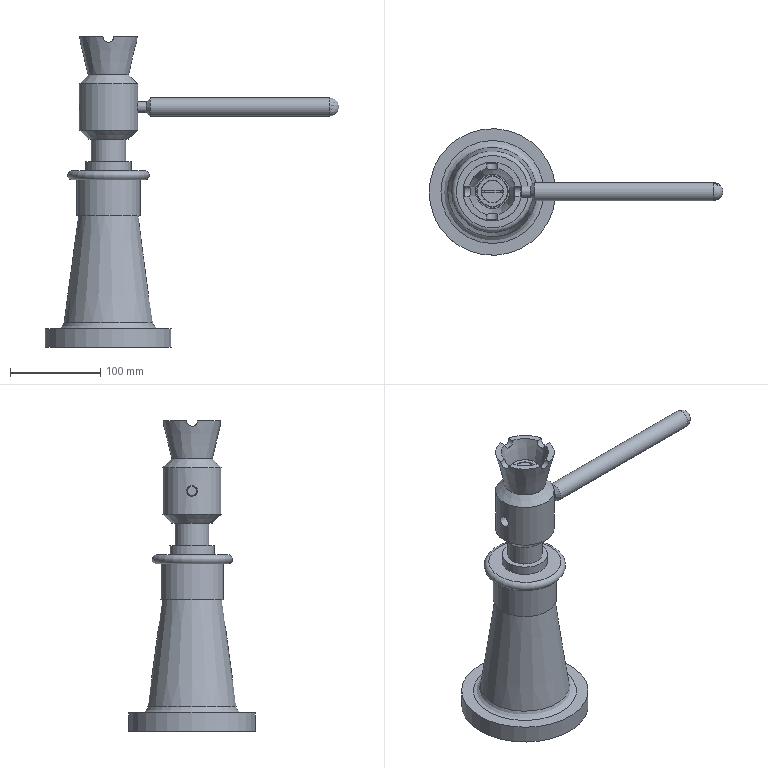Assembly | NX | mm | 7 component files | 7 solids | 67 faces | box 325 x 140 x 343 mm | volume 1154943 mm3 | plane 28 | cylinder 22 | cone 13 | torus 3 | sphere 1 | commonest cylinder face diameters 12 x6 50 x3 38 x2 10.3 x2 20 x1 100 x1 140 x1 70 x1
Bill of materials:
unnamed part 1 | 1 |  | Thick-walled hollow cup tapered like a frustum, wider at the open top. The top rim has four evenly spaced semicircular notches, and the bottom wall has a central through-hole.
unnamed part 2 | 1 |  | Stepped turned pin: a long plain cylindrical shank with a larger cylindrical collar or head that has chamfered edges on both sides. The head has a small radial cross-hole, and a small cylindrical spigot sticks out from the top face.
unnamed part 3 | 1 |  | Slender stepped cylindrical rod: a short smaller-diameter section at one end, a short chamfer or step, then a longer main body that ends in a rounded, roughly hemispherical tip.
unnamed part 4 | 1 |  | Flanged tubular bushing or grommet: a straight cylindrical sleeve with a central through-bore and a thin circular flange with rounded edges around its middle.
unnamed part 5 | 1 |  | Hollow tapered body standing on a flat circular base flange. A conical frustum rises from the flange with a fillet at its root and steps into a short cylindrical neck at the top. A through-bore runs along the axis.
unnamed part 6 | 1 |  | Slotted countersunk-head screw-like part: a conical flat-top head with a straight slot across it, a plain cylindrical shank, and a chamfered tip.
unnamed part 7 | 1 |  | Countersunk ring or cup washer: a flat cylindrical ring with a conical countersink on one face that leads into a central through-hole. The outer top edge is slightly rounded.
Mates:
1. fix | Body 1 component
2. touch align | Nut 1 face | Body 1 face
3. touch align | Body 1 face | Nut 1 face
4. touch align | Screw_Spindle 1 face | Nut 1 face
5. distance | Nut 1 face | Screw_Spindle 1 face
6. touch align | Cap 1 face | Screw_Spindle 1 face
7. touch align | Screw_Spindle 1 face | Cap 1 face
8. touch align | Sp_Washer 1 face | Cap 1 face
9. touch align | Screw_Spindle 1 face | Sp_Washer 1 face
10. touch align | Counter_Sunk_Screw 1 face | Sp_Washer 1 face
11. touch align | Sp_Washer 1 face | Counter_Sunk_Screw 1 face
12. touch align | Tommy_Bar 1 face | Screw_Spindle 1 face